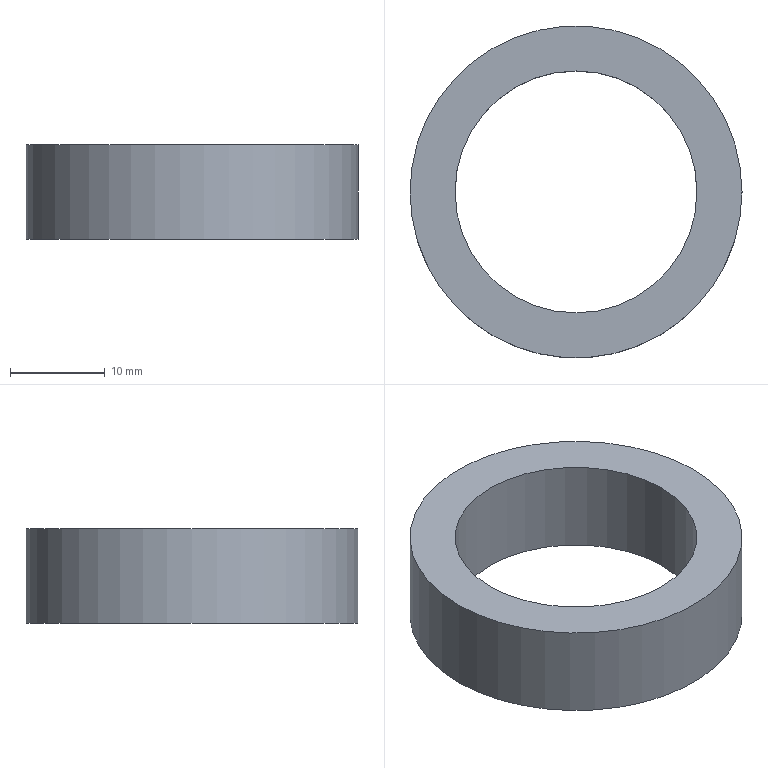Component | NX | SHAFT_SLEEVE_2 | 1 solid | 4 faces | box 35 x 35 x 10 mm | volume 4514 mm3 | cylinder 2 | plane 2 | commonest cylinder face diameters 35 x1 25.5 x1
STEP:
#1=CARTESIAN_POINT('',(0.,0.,0.));
#2=DIRECTION('',(0.,0.,1.));
#3=DIRECTION('',(1.,0.,0.));
#4=AXIS2_PLACEMENT_3D('',#1,#2,#3);
#5=CARTESIAN_POINT('',(-406.675,308.181,-675.));
#6=VERTEX_POINT('',#5);
#7=CARTESIAN_POINT('',(-424.175,308.181,-675.));
#8=DIRECTION('',(0.,0.,1.));
#9=DIRECTION('',(1.,0.,0.));
#10=AXIS2_PLACEMENT_3D('',#7,#8,#9);
#11=CIRCLE('',#10,17.5);
#12=CARTESIAN_POINT('',(-424.175,308.181,-675.));
#13=DIRECTION('',(0.,0.,-1.));
#14=DIRECTION('',(-1.,0.,0.));
#15=AXIS2_PLACEMENT_3D('',#12,#13,#14);
#16=CYLINDRICAL_SURFACE('',#15,17.5);
#17=CARTESIAN_POINT('',(9.425,0.));
#18=DIRECTION('',(-1.,0.));
#19=VECTOR('',#18,1.);
#20=LINE('',#17,#19);
#21=(GEOMETRIC_REPRESENTATION_CONTEXT(2)PARAMETRIC_REPRESENTATION_CONTEXT()REPRESENTATION_CONTEXT('',''));
#22=DEFINITIONAL_REPRESENTATION('',(#20),#21);
#23=PCURVE('',#16,#22);
#24=CARTESIAN_POINT('',(-424.175,308.181,-675.));
#25=DIRECTION('',(0.,0.,1.));
#26=DIRECTION('',(1.,0.,0.));
#27=AXIS2_PLACEMENT_3D('',#24,#25,#26);
#28=PLANE('',#27);
#29=CARTESIAN_POINT('',(0.,0.));
#30=DIRECTION('',(1.,0.));
#31=AXIS2_PLACEMENT_2D('',#29,#30);
#32=CIRCLE('',#31,17.5);
#33=(GEOMETRIC_REPRESENTATION_CONTEXT(2)PARAMETRIC_REPRESENTATION_CONTEXT()REPRESENTATION_CONTEXT('',''));
#34=DEFINITIONAL_REPRESENTATION('',(#32),#33);
#35=PCURVE('',#28,#34);
#36=SURFACE_CURVE('',#11,(#23,#35),.PCURVE_S1.);
#37=EDGE_CURVE('',#6,#6,#36,.T.);
#38=ORIENTED_EDGE('',*,*,#37,.F.);
#39=CARTESIAN_POINT('',(-406.675,308.181,-685.));
#40=VERTEX_POINT('',#39);
#41=CARTESIAN_POINT('',(-406.675,308.181,-675.));
#42=CARTESIAN_POINT('',(-406.675,308.181,-685.));
#43=B_SPLINE_CURVE_WITH_KNOTS('',1,(#41,#42),.UNSPECIFIED.,.F.,.F.,(2,2),(0.,10.),.PIECEWISE_BEZIER_KNOTS.);
#44=CARTESIAN_POINT('',(9.425,0.));
#45=DIRECTION('',(0.,1.));
#46=VECTOR('',#45,1.);
#47=LINE('',#44,#46);
#48=(GEOMETRIC_REPRESENTATION_CONTEXT(2)PARAMETRIC_REPRESENTATION_CONTEXT()REPRESENTATION_CONTEXT('',''));
#49=DEFINITIONAL_REPRESENTATION('',(#47),#48);
#50=PCURVE('',#16,#49);
#51=CARTESIAN_POINT('',(3.142,0.));
#52=DIRECTION('',(0.,1.));
#53=VECTOR('',#52,1.);
#54=LINE('',#51,#53);
#55=(GEOMETRIC_REPRESENTATION_CONTEXT(2)PARAMETRIC_REPRESENTATION_CONTEXT()REPRESENTATION_CONTEXT('',''));
#56=DEFINITIONAL_REPRESENTATION('',(#54),#55);
#57=PCURVE('',#16,#56);
#58=SEAM_CURVE('',#43,(#50,#57),.PCURVE_S1.);
#59=EDGE_CURVE('',#6,#40,#58,.T.);
#60=ORIENTED_EDGE('',*,*,#59,.T.);
#61=CARTESIAN_POINT('',(-424.175,308.181,-685.));
#62=DIRECTION('',(0.,0.,1.));
#63=DIRECTION('',(1.,0.,0.));
#64=AXIS2_PLACEMENT_3D('',#61,#62,#63);
#65=CIRCLE('',#64,17.5);
#66=CARTESIAN_POINT('',(9.425,10.));
#67=DIRECTION('',(-1.,0.));
#68=VECTOR('',#67,1.);
#69=LINE('',#66,#68);
#70=(GEOMETRIC_REPRESENTATION_CONTEXT(2)PARAMETRIC_REPRESENTATION_CONTEXT()REPRESENTATION_CONTEXT('',''));
#71=DEFINITIONAL_REPRESENTATION('',(#69),#70);
#72=PCURVE('',#16,#71);
#73=CARTESIAN_POINT('',(-424.175,308.181,-685.));
#74=DIRECTION('',(0.,0.,1.));
#75=DIRECTION('',(1.,0.,0.));
#76=AXIS2_PLACEMENT_3D('',#73,#74,#75);
#77=PLANE('',#76);
#78=CARTESIAN_POINT('',(0.,0.));
#79=DIRECTION('',(1.,0.));
#80=AXIS2_PLACEMENT_2D('',#78,#79);
#81=CIRCLE('',#80,17.5);
#82=(GEOMETRIC_REPRESENTATION_CONTEXT(2)PARAMETRIC_REPRESENTATION_CONTEXT()REPRESENTATION_CONTEXT('',''));
#83=DEFINITIONAL_REPRESENTATION('',(#81),#82);
#84=PCURVE('',#77,#83);
#85=SURFACE_CURVE('',#65,(#72,#84),.PCURVE_S1.);
#86=EDGE_CURVE('',#40,#40,#85,.T.);
#87=ORIENTED_EDGE('',*,*,#86,.T.);
#88=ORIENTED_EDGE('',*,*,#59,.F.);
#89=EDGE_LOOP('',(#38,#60,#87,#88));
#90=FACE_BOUND('',#89,.T.);
#91=ADVANCED_FACE('',(#90),#16,.T.);
#92=CARTESIAN_POINT('',(-411.425,308.181,-675.));
#93=VERTEX_POINT('',#92);
#94=CARTESIAN_POINT('',(-424.175,308.181,-675.));
#95=DIRECTION('',(0.,0.,1.));
#96=DIRECTION('',(1.,0.,0.));
#97=AXIS2_PLACEMENT_3D('',#94,#95,#96);
#98=CIRCLE('',#97,12.75);
#99=CARTESIAN_POINT('',(-424.175,308.181,-675.));
#100=DIRECTION('',(0.,0.,-1.));
#101=DIRECTION('',(-1.,0.,0.));
#102=AXIS2_PLACEMENT_3D('',#99,#100,#101);
#103=CYLINDRICAL_SURFACE('',#102,12.75);
#104=CARTESIAN_POINT('',(9.425,0.));
#105=DIRECTION('',(-1.,0.));
#106=VECTOR('',#105,1.);
#107=LINE('',#104,#106);
#108=(GEOMETRIC_REPRESENTATION_CONTEXT(2)PARAMETRIC_REPRESENTATION_CONTEXT()REPRESENTATION_CONTEXT('',''));
#109=DEFINITIONAL_REPRESENTATION('',(#107),#108);
#110=PCURVE('',#103,#109);
#111=CARTESIAN_POINT('',(0.,0.));
#112=DIRECTION('',(1.,0.));
#113=AXIS2_PLACEMENT_2D('',#111,#112);
#114=CIRCLE('',#113,12.75);
#115=(GEOMETRIC_REPRESENTATION_CONTEXT(2)PARAMETRIC_REPRESENTATION_CONTEXT()REPRESENTATION_CONTEXT('',''));
#116=DEFINITIONAL_REPRESENTATION('',(#114),#115);
#117=PCURVE('',#28,#116);
#118=SURFACE_CURVE('',#98,(#110,#117),.PCURVE_S1.);
#119=EDGE_CURVE('',#93,#93,#118,.T.);
#120=ORIENTED_EDGE('',*,*,#119,.F.);
#121=CARTESIAN_POINT('',(-411.425,308.181,-685.));
#122=VERTEX_POINT('',#121);
#123=CARTESIAN_POINT('',(-411.425,308.181,-675.));
#124=CARTESIAN_POINT('',(-411.425,308.181,-685.));
#125=B_SPLINE_CURVE_WITH_KNOTS('',1,(#123,#124),.UNSPECIFIED.,.F.,.F.,(2,2),(0.,10.),.PIECEWISE_BEZIER_KNOTS.);
#126=CARTESIAN_POINT('',(9.425,0.));
#127=DIRECTION('',(0.,1.));
#128=VECTOR('',#127,1.);
#129=LINE('',#126,#128);
#130=(GEOMETRIC_REPRESENTATION_CONTEXT(2)PARAMETRIC_REPRESENTATION_CONTEXT()REPRESENTATION_CONTEXT('',''));
#131=DEFINITIONAL_REPRESENTATION('',(#129),#130);
#132=PCURVE('',#103,#131);
#133=CARTESIAN_POINT('',(3.142,0.));
#134=DIRECTION('',(0.,1.));
#135=VECTOR('',#134,1.);
#136=LINE('',#133,#135);
#137=(GEOMETRIC_REPRESENTATION_CONTEXT(2)PARAMETRIC_REPRESENTATION_CONTEXT()REPRESENTATION_CONTEXT('',''));
#138=DEFINITIONAL_REPRESENTATION('',(#136),#137);
#139=PCURVE('',#103,#138);
#140=SEAM_CURVE('',#125,(#132,#139),.PCURVE_S1.);
#141=EDGE_CURVE('',#93,#122,#140,.T.);
#142=ORIENTED_EDGE('',*,*,#141,.T.);
#143=CARTESIAN_POINT('',(-424.175,308.181,-685.));
#144=DIRECTION('',(0.,0.,1.));
#145=DIRECTION('',(1.,0.,0.));
#146=AXIS2_PLACEMENT_3D('',#143,#144,#145);
#147=CIRCLE('',#146,12.75);
#148=CARTESIAN_POINT('',(9.425,10.));
#149=DIRECTION('',(-1.,0.));
#150=VECTOR('',#149,1.);
#151=LINE('',#148,#150);
#152=(GEOMETRIC_REPRESENTATION_CONTEXT(2)PARAMETRIC_REPRESENTATION_CONTEXT()REPRESENTATION_CONTEXT('',''));
#153=DEFINITIONAL_REPRESENTATION('',(#151),#152);
#154=PCURVE('',#103,#153);
#155=CARTESIAN_POINT('',(0.,0.));
#156=DIRECTION('',(1.,0.));
#157=AXIS2_PLACEMENT_2D('',#155,#156);
#158=CIRCLE('',#157,12.75);
#159=(GEOMETRIC_REPRESENTATION_CONTEXT(2)PARAMETRIC_REPRESENTATION_CONTEXT()REPRESENTATION_CONTEXT('',''));
#160=DEFINITIONAL_REPRESENTATION('',(#158),#159);
#161=PCURVE('',#77,#160);
#162=SURFACE_CURVE('',#147,(#154,#161),.PCURVE_S1.);
#163=EDGE_CURVE('',#122,#122,#162,.T.);
#164=ORIENTED_EDGE('',*,*,#163,.T.);
#165=ORIENTED_EDGE('',*,*,#141,.F.);
#166=EDGE_LOOP('',(#120,#142,#164,#165));
#167=FACE_BOUND('',#166,.F.);
#168=ADVANCED_FACE('',(#167),#103,.F.);
#169=ORIENTED_EDGE('',*,*,#37,.T.);
#170=EDGE_LOOP('',(#169));
#171=FACE_BOUND('',#170,.T.);
#172=ORIENTED_EDGE('',*,*,#119,.F.);
#173=EDGE_LOOP('',(#172));
#174=FACE_BOUND('',#173,.T.);
#175=ADVANCED_FACE('',(#171,#174),#28,.T.);
#176=ORIENTED_EDGE('',*,*,#86,.F.);
#177=EDGE_LOOP('',(#176));
#178=FACE_BOUND('',#177,.T.);
#179=ORIENTED_EDGE('',*,*,#163,.T.);
#180=EDGE_LOOP('',(#179));
#181=FACE_BOUND('',#180,.T.);
#182=ADVANCED_FACE('',(#178,#181),#77,.F.);
#183=CLOSED_SHELL('',(#91,#168,#175,#182));
#184=MANIFOLD_SOLID_BREP('',#183);
#185=(LENGTH_UNIT()NAMED_UNIT(*)SI_UNIT(.MILLI.,.METRE.));
#186=UNCERTAINTY_MEASURE_WITH_UNIT(LENGTH_MEASURE(0.00001),#185,'','');
#187=(NAMED_UNIT(*)PLANE_ANGLE_UNIT()SI_UNIT($,.RADIAN.));
#188=(NAMED_UNIT(*)SI_UNIT($,.STERADIAN.)SOLID_ANGLE_UNIT());
#189=(GEOMETRIC_REPRESENTATION_CONTEXT(3)GLOBAL_UNCERTAINTY_ASSIGNED_CONTEXT((#186))GLOBAL_UNIT_ASSIGNED_CONTEXT((#185,#187,#188))REPRESENTATION_CONTEXT('',''));
#190=ADVANCED_BREP_SHAPE_REPRESENTATION('',(#4,#184),#189);